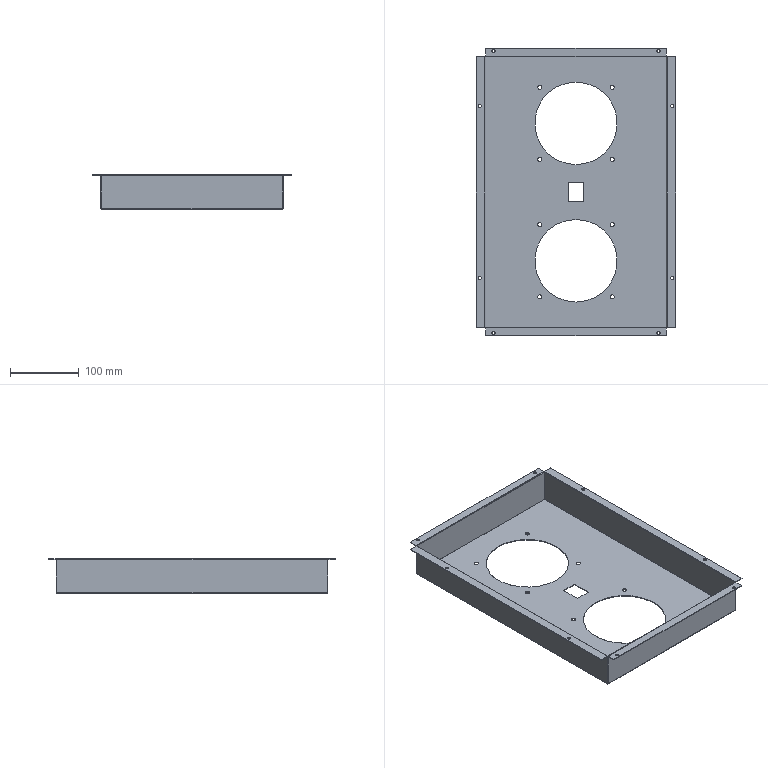Component | SolidWorks | FanMountingPlate-1 | 1 solid | 110 faces | volume 160634 mm3 | plane 58 | cylinder 52 | commonest cylinder face diameters 6.1 x16 4.5 x16 0.02 x8 2.02 x8 120 x4